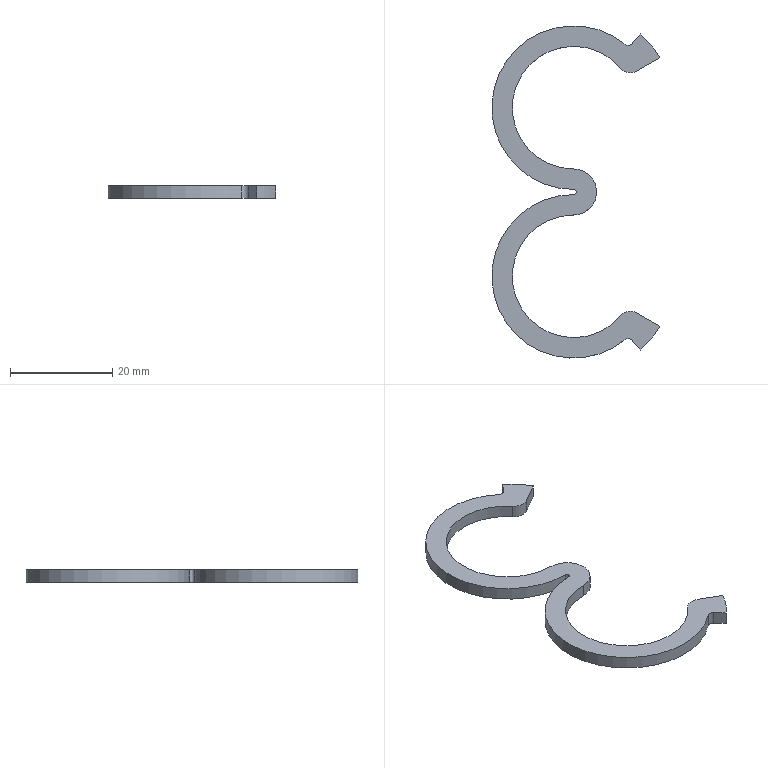Component | NX | 12 | 1 solid | 18 faces | volume 1343 mm3 | cylinder 12 | plane 6 | commonest cylinder face diameters 39 x2 2 x2 32 x2 5 x2 24 x2 1 x1 9 x1